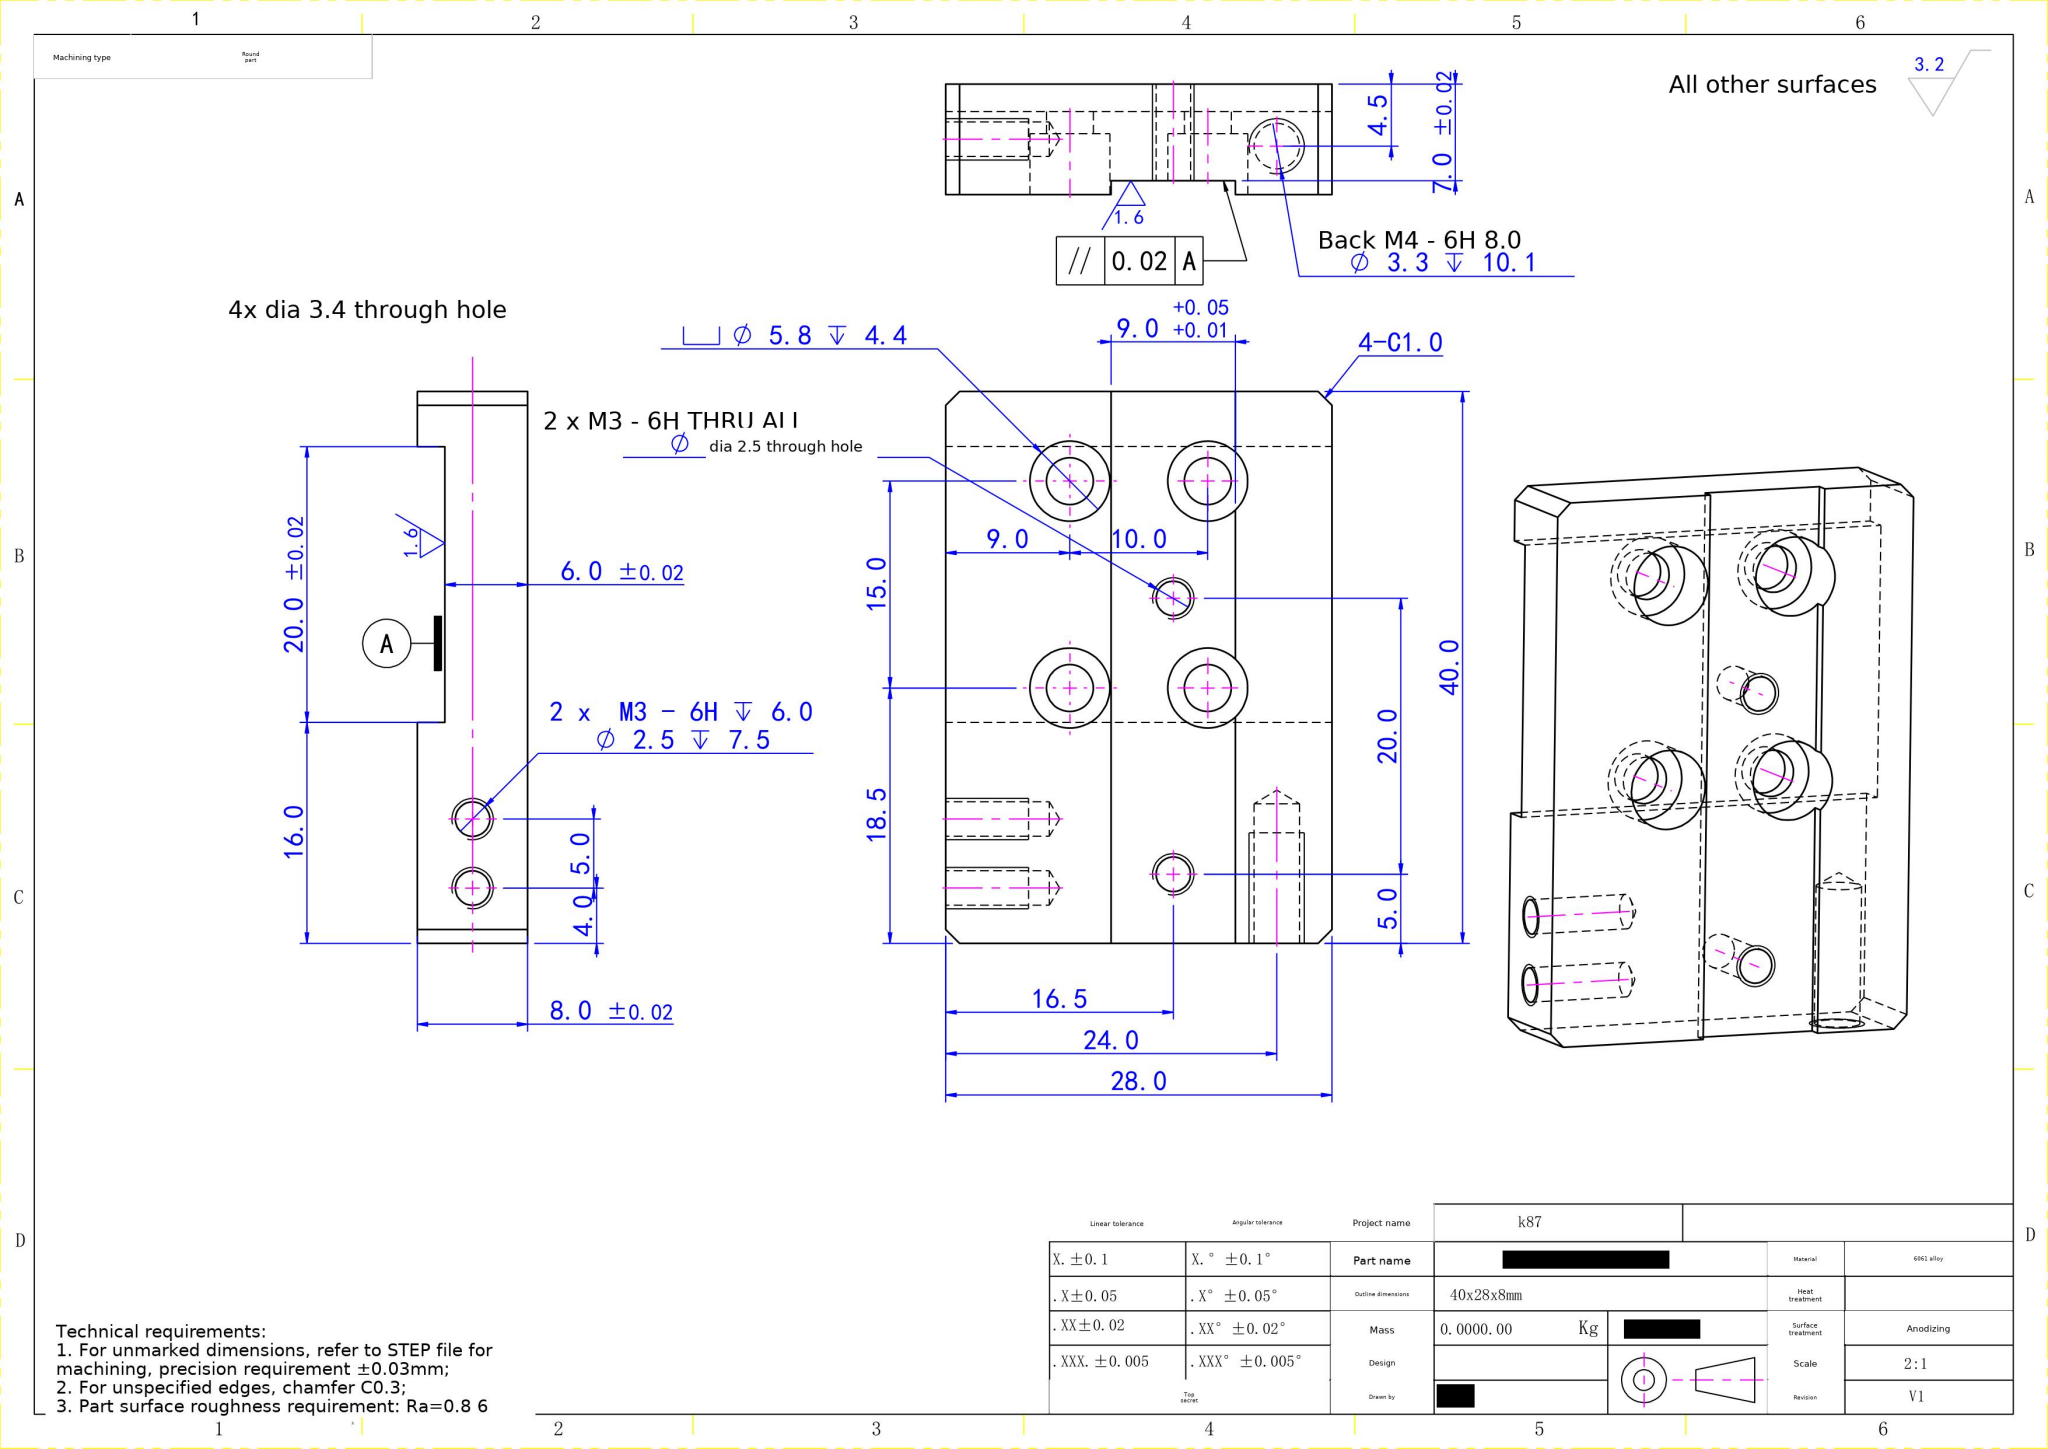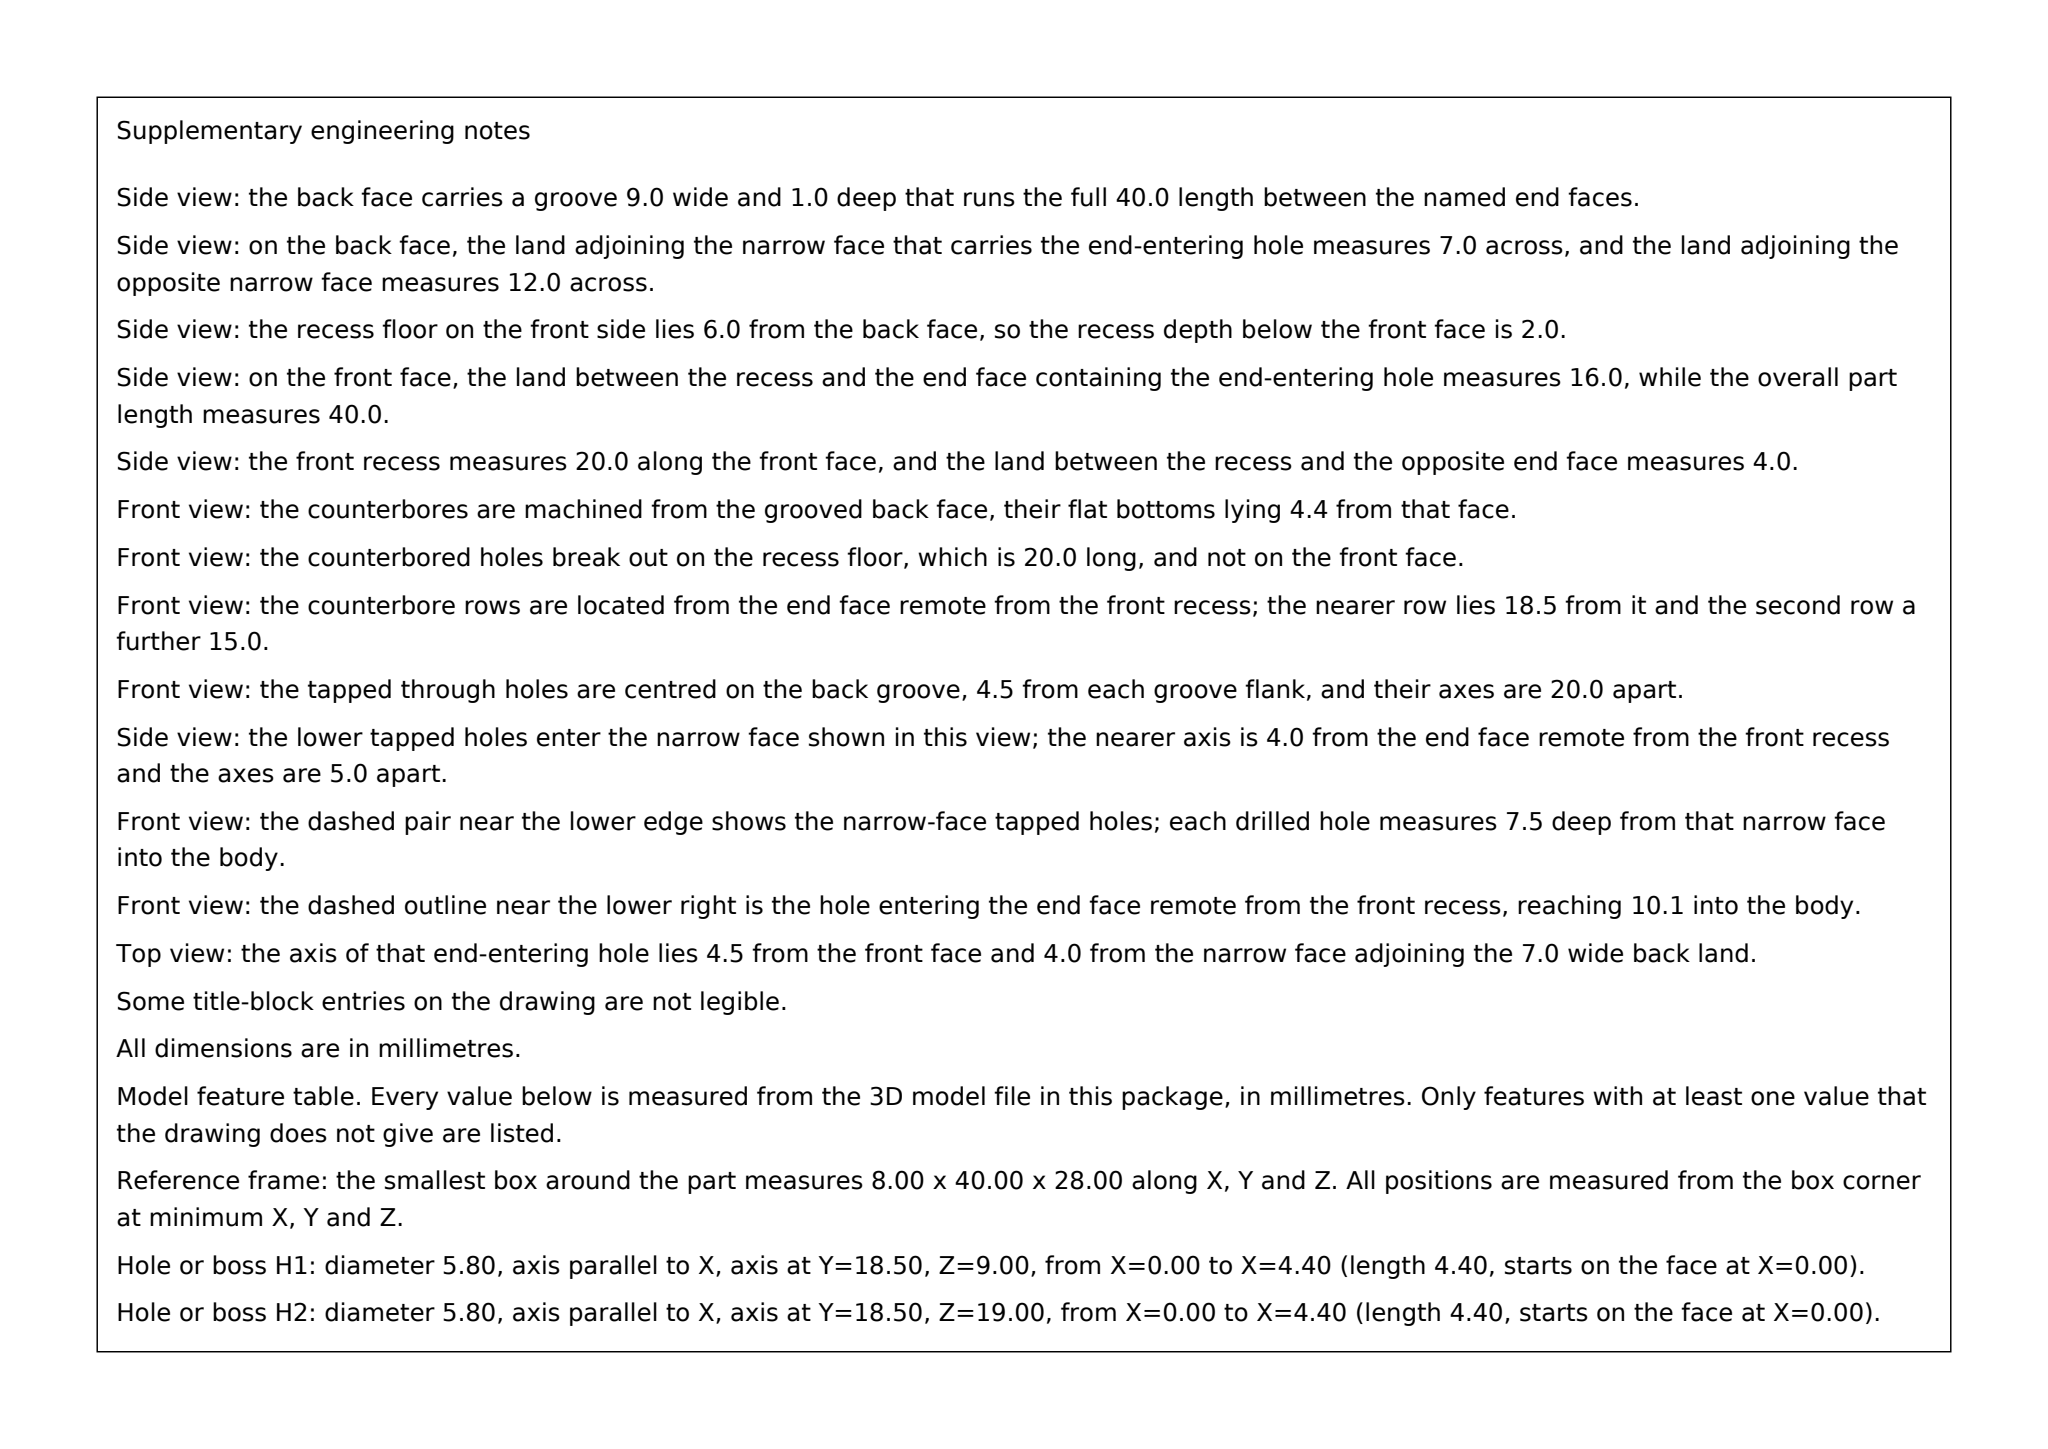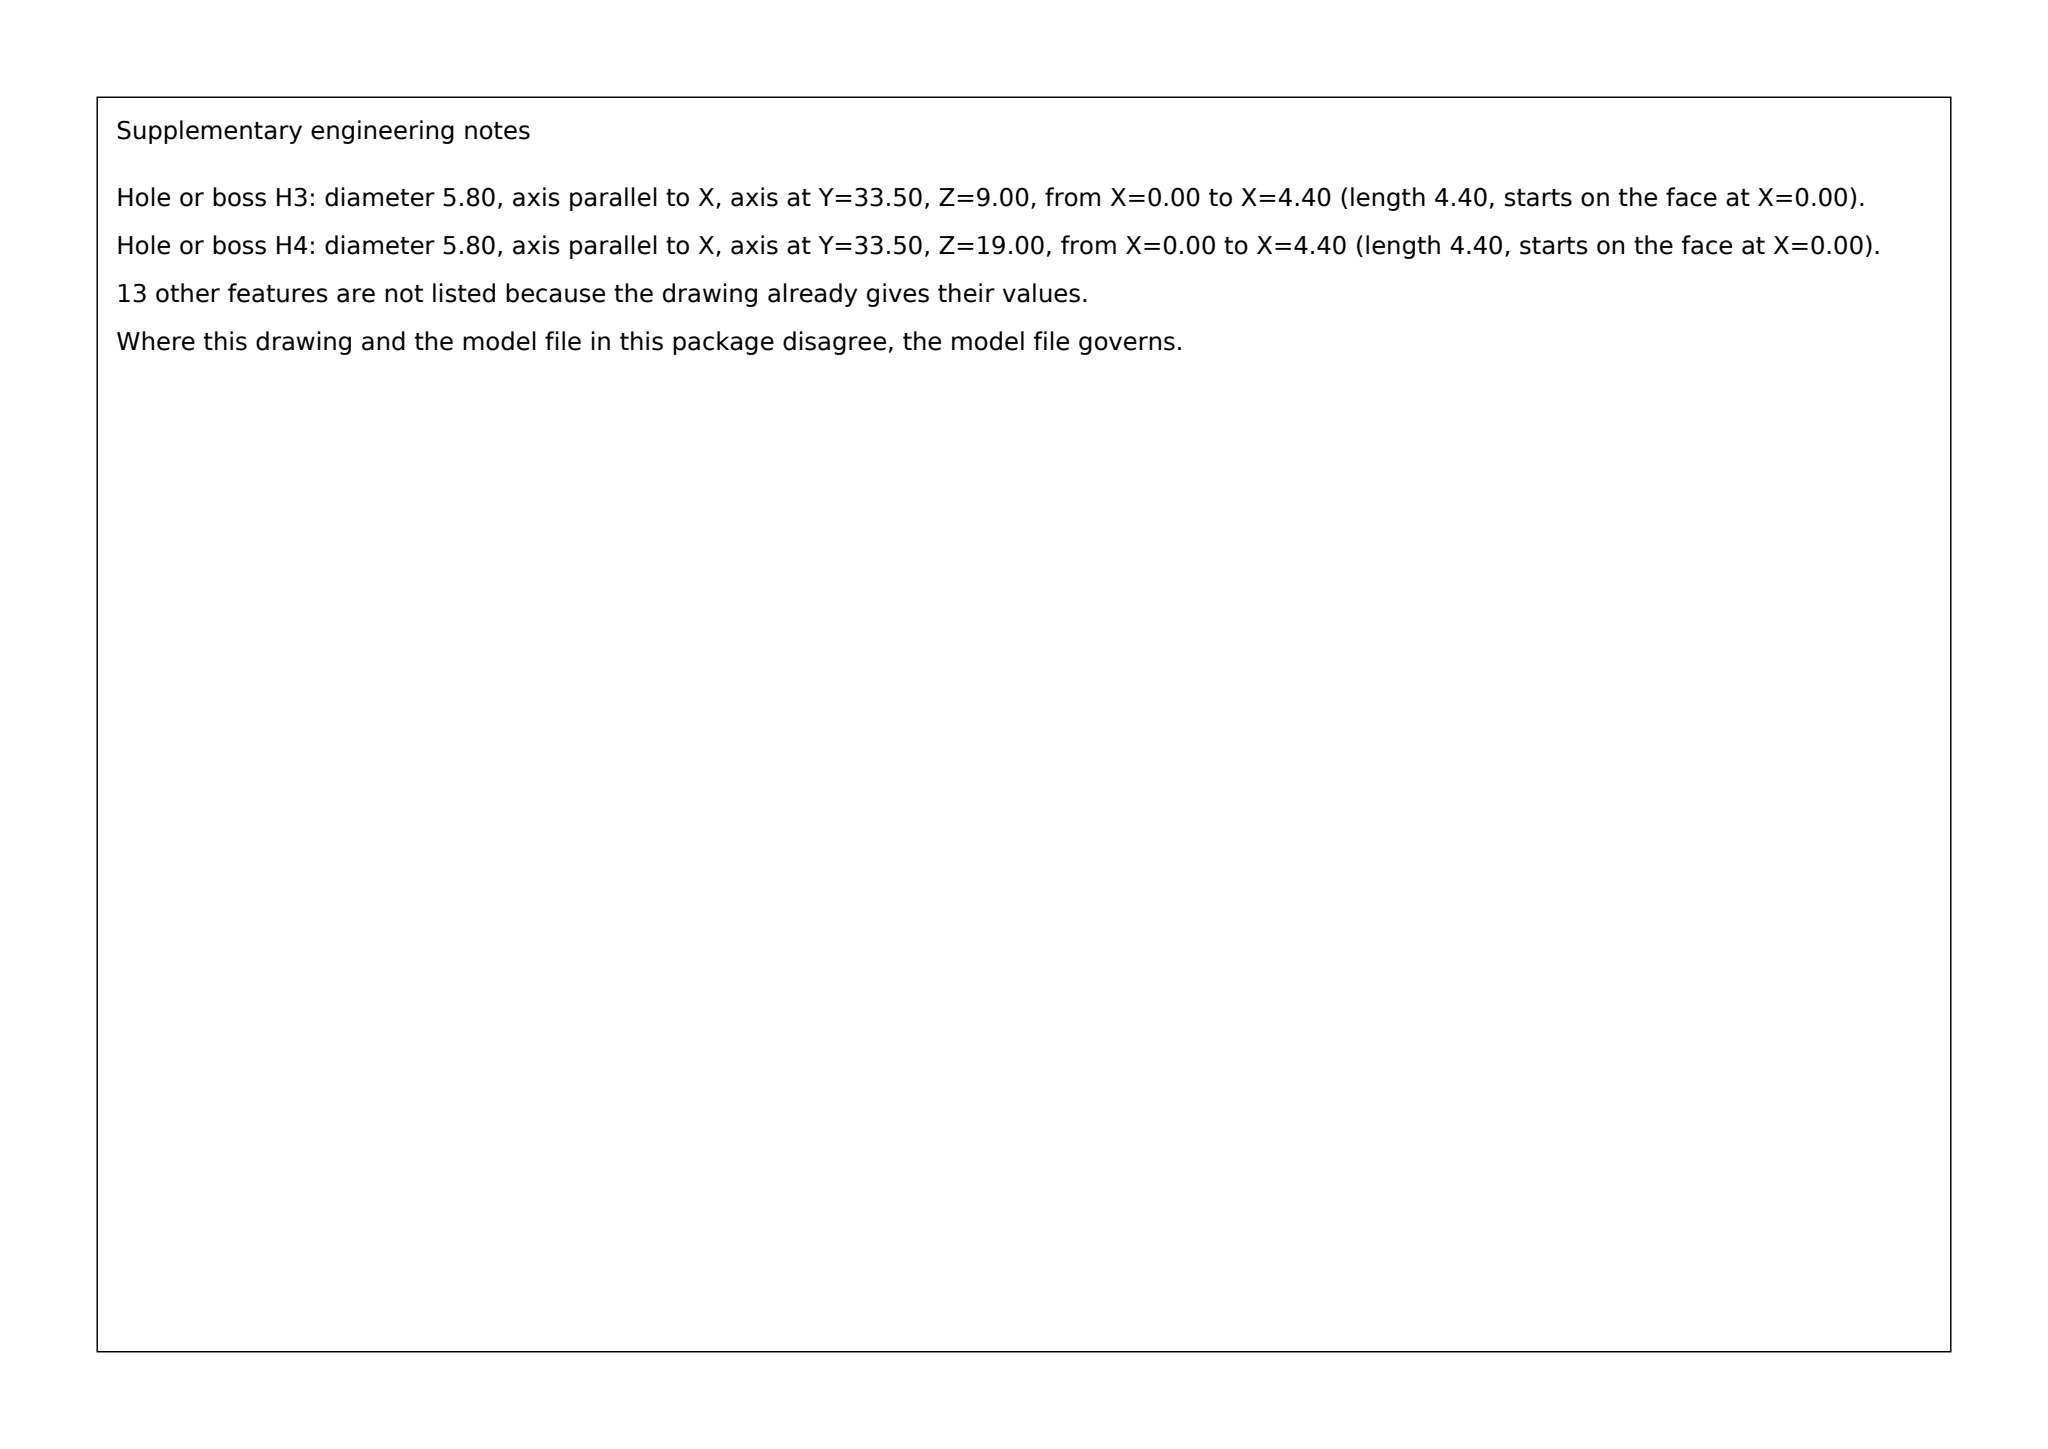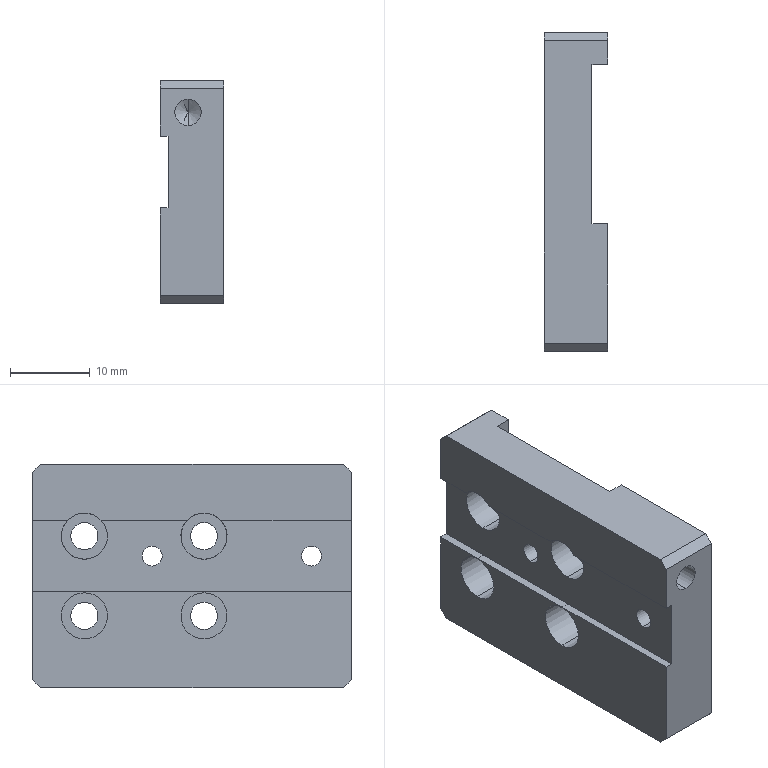Part | SolidWorks | mm | material 6061 alloy | 1 solid | 56 faces | box 8 x 40 x 28 mm | volume 6764 mm3 | cylinder 26 | plane 24 | cone 6 | commonest cylinder face diameters 2.5 x8 5.8 x8 3.4 x8 3.3 x2
Drawing notes:
BACK GROOVE 9.0(+.05/+.01) W x 1.0 DP, FULL 40 LG, 12.0 FROM LH EDGE | from the solid: Plane x=1.0 spans z 12.0-21.0 (9.0 wide), y 0-40 full length; back face x=0.0 gives 1.0 depth; groove near edge at z=12.0 from z=0 (left edge of front view)
2 x M3-6H THRU ALL, Ø2.5 TAP DRILL THRU (NO PLAIN Ø2.5 HOLE) | from the solid: Ø2.5 holes on x axis at (y=25.0, z=16.5) x1.0-6.0 and (y=5.0, z=16.5) x1.0-8.0: both break through full material, no drill-point cone
BACK FACE: M4-6H DP 8.0, Ø3.3 DP 10.1 | from the solid: Ø3.3 hole on y axis at x=3.5, z=24.0, from y=0.0 to 10.1 (drill depth 10.1) with 118° point